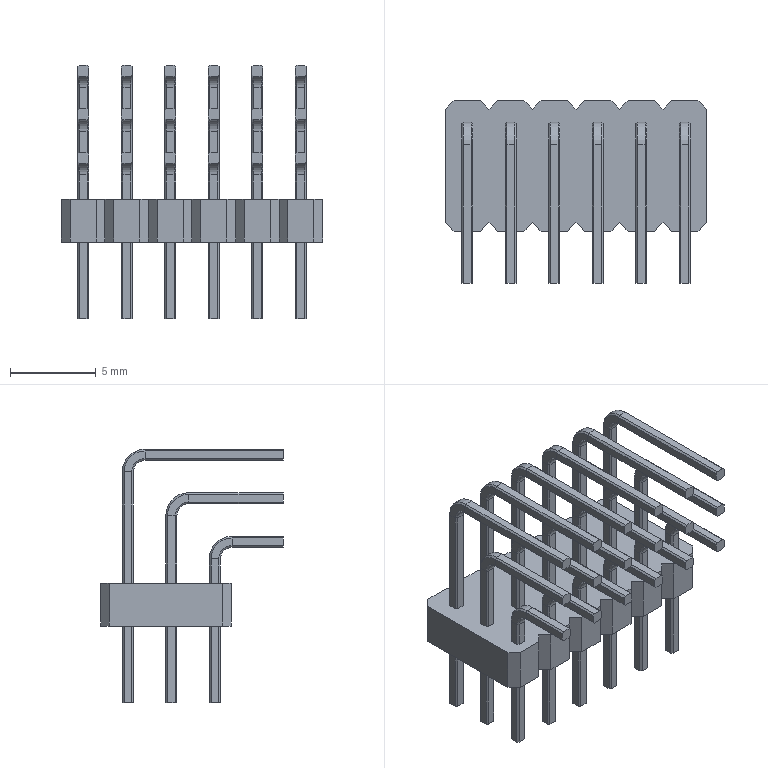Component | SolidWorks | Assembly 1-1_13.Electrical unit 2-2 | 1 solid | 652 faces | box 15.24 x 10.68 x 14.81 mm | volume 395 mm3 | plane 544 | cone 72 | cylinder 36 | commonest cylinder face diameters 1.35 x18 2.65 x18
build123d program:
from build123d import *

# Parameters (mm, degrees)
BOSS_EXTRUDE1_DEPTH = 2.5
LPATTERN1_COUNT     = 6
LPATTERN1_PITCH     = 2.54


with BuildPart() as part:
    # Sweep1: sweep along a path in Sketch2
    with BuildLine(Plane.XY) as sweep1_path:
        Line((5.08, 0), (5.08, 3))
        ThreePointArc((5.08, 3), (5.373, 3.707), (6.08, 4))
        Line((6.08, 4), (14.48, 4))
    # Sketch1 → Sweep1 (sweep)
    with BuildSketch(Plane(origin=(0, 0, 0), x_dir=(1, 0, 0), z_dir=(0, 1, 0))):
        Polygon((4.855, 0.325), (5.305, 0.325), (5.405, 0.225), (5.405, -0.225), (5.305, -0.325), (4.855, -0.325), (4.755, -0.225), (4.755, 0.225), align=None)
    sweep(path=sweep1_path.line)



with BuildPart() as body_2:
    # Sweep2: sweep along a path in Sketch2_3
    with BuildLine(Plane.XY) as sweep2_path:
        Line((2.54, 0), (2.54, 5.54))
        ThreePointArc((2.54, 5.54), (2.833, 6.247), (3.54, 6.54))
        Line((3.54, 6.54), (14.48, 6.54))
    # Sketch1_3 → Sweep2 (sweep)
    with BuildSketch(Plane(origin=(0, 0, 0), x_dir=(1, 0, 0), z_dir=(0, 1, 0))):
        Polygon((2.315, 0.325), (2.765, 0.325), (2.865, 0.225), (2.865, -0.225), (2.765, -0.325), (2.315, -0.325), (2.215, -0.225), (2.215, 0.225), align=None)
    sweep(path=sweep2_path.line)


with BuildPart() as body_3:
    # Sweep3: sweep along a path in Sketch2_4
    with BuildLine(Plane.XY) as sweep3_path:
        Line((0, 0), (0, 8.08))
        ThreePointArc((0, 8.08), (0.2929, 8.787), (1, 9.08))
        Line((1, 9.08), (14.48, 9.08))
    # Sketch1_4 → Sweep3 (sweep)
    with BuildSketch(Plane(origin=(0, 0, 0), x_dir=(1, 0, 0), z_dir=(0, 1, 0))):
        Polygon((-0.325, 0.225), (-0.225, 0.325), (0.225, 0.325), (0.325, 0.225), (0.325, -0.225), (0.225, -0.325), (-0.225, -0.325), (-0.325, -0.225), align=None)
    sweep(path=sweep3_path.line)


with BuildPart() as part_1:
    add(part.part)

    add(body_2.part)  # Boss-Extrude1 merges body 2

    add(body_3.part)  # Boss-Extrude1 merges body 3
    # Sketch3 → Boss-Extrude1 (add)
    with BuildSketch(Plane(origin=(7.5, 0, 0), x_dir=(0, 0, -1), z_dir=(1, 0, 0))):
        Polygon((-0.77, 10.675), (0.77, 10.675), (1.27, 10.175), (1.27, 3.555), (0.77, 3.055), (-0.77, 3.055), (-1.27, 3.555), (-1.27, 10.175), align=None)
    extrude(amount=BOSS_EXTRUDE1_DEPTH)


with BuildPart() as lpattern1_1:
    # LPattern1: pattern copy
    add(part_1.part.moved(Location(Vector(0, 0, -1) * (1 * LPATTERN1_PITCH))))


with BuildPart() as lpattern1_2:
    # LPattern1: pattern copy
    add(part_1.part.moved(Location(Vector(0, 0, -1) * (2 * LPATTERN1_PITCH))))


with BuildPart() as lpattern1_3:
    # LPattern1: pattern copy
    add(part_1.part.moved(Location(Vector(0, 0, -1) * (3 * LPATTERN1_PITCH))))


with BuildPart() as lpattern1_4:
    # LPattern1: pattern copy
    add(part_1.part.moved(Location(Vector(0, 0, -1) * (4 * LPATTERN1_PITCH))))


with BuildPart() as lpattern1_5:
    # LPattern1: pattern copy
    add(part_1.part.moved(Location(Vector(0, 0, -1) * (5 * LPATTERN1_PITCH))))


with BuildPart() as part_2:
    add(part_1.part)

    # Combine1: union LPattern1_1, LPattern1_2, LPattern1_3, LPattern1_4, LPattern1_5
    add(lpattern1_1.part)
    add(lpattern1_2.part)
    add(lpattern1_3.part)
    add(lpattern1_4.part)
    add(lpattern1_5.part)


solid = part_2.part

# Placed as in the assembly
solid = solid.moved(Location((3.97, 10.095, -10.8), (0, 90, 0)))